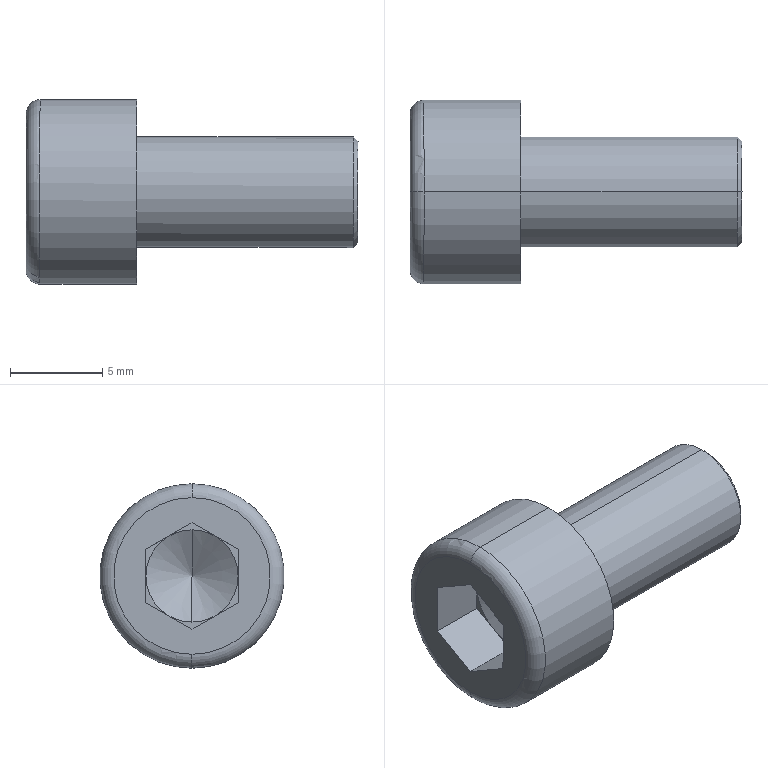Component | SolidWorks | hexagon socket head cap screws gb-88 | 1 solid | 25 faces | box 18.01 x 10 x 10.01 mm | volume 732 mm3 | plane 15 | cone 4 | cylinder 4 | torus 2 | commonest cylinder face diameters 6 x2 10 x2
STEP:
#1=COLOUR_RGB('',0.7922,0.8196,0.9333);
#2=FILL_AREA_STYLE_COLOUR('',#1);
#3=FILL_AREA_STYLE('',(#2));
#4=SURFACE_STYLE_FILL_AREA(#3);
#5=SURFACE_SIDE_STYLE('',(#4));
#6=SURFACE_STYLE_USAGE(.BOTH.,#5);
#7=PRESENTATION_STYLE_ASSIGNMENT((#6));
#8=CARTESIAN_POINT('',(-2.934,36.006,44.762));
#9=VERTEX_POINT('',#8);
#10=CARTESIAN_POINT('',(-2.933,36.006,44.978));
#11=VERTEX_POINT('',#10);
#12=CARTESIAN_POINT('',(-2.933,36.006,44.87));
#13=DIRECTION('',(1.,0.,-0.00108));
#14=DIRECTION('',(-0.00108,0.,-1.));
#15=AXIS2_PLACEMENT_3D('',#12,#13,#14);
#16=CIRCLE('',#15,0.1083);
#17=EDGE_CURVE('',#9,#11,#16,.T.);
#18=ORIENTED_EDGE('',*,*,#17,.F.);
#19=CARTESIAN_POINT('',(-2.943,36.006,44.752));
#20=VERTEX_POINT('',#19);
#21=CARTESIAN_POINT('',(-2.934,36.006,44.762));
#22=DIRECTION('',(-0.7079,0.,-0.7063));
#23=VECTOR('',#22,39.37);
#24=LINE('',#21,#23);
#25=EDGE_CURVE('',#9,#20,#24,.T.);
#26=ORIENTED_EDGE('',*,*,#25,.T.);
#27=CARTESIAN_POINT('',(-2.943,36.006,44.988));
#28=VERTEX_POINT('',#27);
#29=CARTESIAN_POINT('',(-2.943,36.006,44.87));
#30=DIRECTION('',(-1.,-0.,0.00108));
#31=DIRECTION('',(-0.00108,0.,-1.));
#32=AXIS2_PLACEMENT_3D('',#29,#30,#31);
#33=CIRCLE('',#32,0.1181);
#34=EDGE_CURVE('',#28,#20,#33,.T.);
#35=ORIENTED_EDGE('',*,*,#34,.F.);
#36=CARTESIAN_POINT('',(-2.933,36.006,44.978));
#37=DIRECTION('',(-0.7063,-0.,0.7079));
#38=VECTOR('',#37,39.37);
#39=LINE('',#36,#38);
#40=EDGE_CURVE('',#11,#28,#39,.T.);
#41=ORIENTED_EDGE('',*,*,#40,.F.);
#42=EDGE_LOOP('',(#18,#26,#35,#41));
#43=FACE_OUTER_BOUND('',#42,.T.);
#44=CARTESIAN_POINT('',(-2.933,36.006,44.87));
#45=DIRECTION('',(-1.,-0.,0.00108));
#46=DIRECTION('',(0.00108,-0.,1.));
#47=AXIS2_PLACEMENT_3D('',#44,#45,#46);
#48=CONICAL_SURFACE('',#47,0.1083,0.7854);
#49=ADVANCED_FACE('',(#43),#48,.T.);
#50=CARTESIAN_POINT('',(-3.642,36.006,45.038));
#51=VERTEX_POINT('',#50);
#52=CARTESIAN_POINT('',(-3.642,36.006,44.703));
#53=VERTEX_POINT('',#52);
#54=CARTESIAN_POINT('',(-3.642,36.006,44.871));
#55=DIRECTION('',(-1.,-0.,0.00108));
#56=DIRECTION('',(-0.00108,0.,-1.));
#57=AXIS2_PLACEMENT_3D('',#54,#55,#56);
#58=CIRCLE('',#57,0.1673);
#59=EDGE_CURVE('',#51,#53,#58,.T.);
#60=ORIENTED_EDGE('',*,*,#59,.F.);
#61=CARTESIAN_POINT('',(-3.612,36.006,45.068));
#62=VERTEX_POINT('',#61);
#63=CARTESIAN_POINT('',(-3.612,36.006,45.038));
#64=DIRECTION('',(0.,1.,0.));
#65=DIRECTION('',(0.,-0.,1.));
#66=AXIS2_PLACEMENT_3D('',#63,#64,#65);
#67=CIRCLE('',#66,0.02953);
#68=EDGE_CURVE('',#51,#62,#67,.T.);
#69=ORIENTED_EDGE('',*,*,#68,.T.);
#70=CARTESIAN_POINT('',(-3.613,36.006,44.674));
#71=VERTEX_POINT('',#70);
#72=CARTESIAN_POINT('',(-3.613,36.006,44.871));
#73=DIRECTION('',(1.,0.,-0.00108));
#74=DIRECTION('',(-0.00108,0.,-1.));
#75=AXIS2_PLACEMENT_3D('',#72,#73,#74);
#76=CIRCLE('',#75,0.1969);
#77=EDGE_CURVE('',#71,#62,#76,.T.);
#78=ORIENTED_EDGE('',*,*,#77,.F.);
#79=CARTESIAN_POINT('',(-3.613,36.006,44.703));
#80=DIRECTION('',(-0.,-1.,-0.));
#81=DIRECTION('',(0.,0.,-1.));
#82=AXIS2_PLACEMENT_3D('',#79,#80,#81);
#83=CIRCLE('',#82,0.02953);
#84=EDGE_CURVE('',#53,#71,#83,.T.);
#85=ORIENTED_EDGE('',*,*,#84,.F.);
#86=EDGE_LOOP('',(#60,#69,#78,#85));
#87=FACE_OUTER_BOUND('',#86,.T.);
#88=CARTESIAN_POINT('',(-3.613,36.006,44.871));
#89=DIRECTION('',(1.,0.,-0.00108));
#90=DIRECTION('',(-0.00108,0.,-1.));
#91=AXIS2_PLACEMENT_3D('',#88,#89,#90);
#92=TOROIDAL_SURFACE('',#91,0.1673,0.02953);
#93=ADVANCED_FACE('',(#87),#92,.T.);
#94=CARTESIAN_POINT('',(-3.467,36.006,44.871));
#95=VERTEX_POINT('',#94);
#96=CARTESIAN_POINT('',(-3.524,36.006,44.969));
#97=VERTEX_POINT('',#96);
#98=CARTESIAN_POINT('',(-3.524,36.006,44.969));
#99=DIRECTION('',(-0.4991,-0.,0.8666));
#100=VECTOR('',#99,39.37);
#101=LINE('',#98,#100);
#102=EDGE_CURVE('',#95,#97,#101,.T.);
#103=ORIENTED_EDGE('',*,*,#102,.F.);
#104=CARTESIAN_POINT('',(-3.524,36.006,44.772));
#105=VERTEX_POINT('',#104);
#106=CARTESIAN_POINT('',(-3.524,36.006,44.772));
#107=DIRECTION('',(-0.5009,0.,-0.8655));
#108=VECTOR('',#107,39.37);
#109=LINE('',#106,#108);
#110=EDGE_CURVE('',#95,#105,#109,.T.);
#111=ORIENTED_EDGE('',*,*,#110,.T.);
#112=CARTESIAN_POINT('',(-3.524,35.956,44.785));
#113=VERTEX_POINT('',#112);
#114=CARTESIAN_POINT('',(-3.524,36.006,44.871));
#115=DIRECTION('',(-1.,-0.,0.00108));
#116=DIRECTION('',(-0.00108,0.,-1.));
#117=AXIS2_PLACEMENT_3D('',#114,#115,#116);
#118=CIRCLE('',#117,0.09843);
#119=EDGE_CURVE('',#105,#113,#118,.T.);
#120=ORIENTED_EDGE('',*,*,#119,.T.);
#121=CARTESIAN_POINT('',(-3.524,35.907,44.871));
#122=VERTEX_POINT('',#121);
#123=CARTESIAN_POINT('',(-3.524,36.006,44.871));
#124=DIRECTION('',(-1.,-0.,0.00108));
#125=DIRECTION('',(-0.00108,0.,-1.));
#126=AXIS2_PLACEMENT_3D('',#123,#124,#125);
#127=CIRCLE('',#126,0.09843);
#128=EDGE_CURVE('',#113,#122,#127,.T.);
#129=ORIENTED_EDGE('',*,*,#128,.T.);
#130=CARTESIAN_POINT('',(-3.524,35.956,44.956));
#131=VERTEX_POINT('',#130);
#132=CARTESIAN_POINT('',(-3.524,36.006,44.871));
#133=DIRECTION('',(-1.,-0.,0.00108));
#134=DIRECTION('',(-0.00108,0.,-1.));
#135=AXIS2_PLACEMENT_3D('',#132,#133,#134);
#136=CIRCLE('',#135,0.09843);
#137=EDGE_CURVE('',#122,#131,#136,.T.);
#138=ORIENTED_EDGE('',*,*,#137,.T.);
#139=CARTESIAN_POINT('',(-3.524,36.006,44.871));
#140=DIRECTION('',(-1.,-0.,0.00108));
#141=DIRECTION('',(-0.00108,0.,-1.));
#142=AXIS2_PLACEMENT_3D('',#139,#140,#141);
#143=CIRCLE('',#142,0.09843);
#144=EDGE_CURVE('',#131,#97,#143,.T.);
#145=ORIENTED_EDGE('',*,*,#144,.T.);
#146=EDGE_LOOP('',(#103,#111,#120,#129,#138,#145));
#147=FACE_OUTER_BOUND('',#146,.T.);
#148=CARTESIAN_POINT('',(-3.524,36.006,44.871));
#149=DIRECTION('',(-1.,-0.,0.00108));
#150=DIRECTION('',(0.00108,-0.,1.));
#151=AXIS2_PLACEMENT_3D('',#148,#149,#150);
#152=CONICAL_SURFACE('',#151,0.09843,1.047);
#153=ADVANCED_FACE('',(#147),#152,.F.);
#154=ORIENTED_EDGE('',*,*,#34,.T.);
#155=CARTESIAN_POINT('',(-3.406,36.006,44.752));
#156=VERTEX_POINT('',#155);
#157=CARTESIAN_POINT('',(-2.934,36.006,44.752));
#158=DIRECTION('',(-1.,-0.,0.00108));
#159=VECTOR('',#158,39.37);
#160=LINE('',#157,#159);
#161=EDGE_CURVE('',#20,#156,#160,.T.);
#162=ORIENTED_EDGE('',*,*,#161,.T.);
#163=CARTESIAN_POINT('',(-3.406,36.006,44.989));
#164=VERTEX_POINT('',#163);
#165=CARTESIAN_POINT('',(-3.406,36.006,44.871));
#166=DIRECTION('',(1.,0.,-0.00108));
#167=DIRECTION('',(-0.00108,0.,-1.));
#168=AXIS2_PLACEMENT_3D('',#165,#166,#167);
#169=CIRCLE('',#168,0.1181);
#170=EDGE_CURVE('',#156,#164,#169,.T.);
#171=ORIENTED_EDGE('',*,*,#170,.T.);
#172=CARTESIAN_POINT('',(-2.933,36.006,44.988));
#173=DIRECTION('',(-1.,-0.,0.00108));
#174=VECTOR('',#173,39.37);
#175=LINE('',#172,#174);
#176=EDGE_CURVE('',#28,#164,#175,.T.);
#177=ORIENTED_EDGE('',*,*,#176,.F.);
#178=EDGE_LOOP('',(#154,#162,#171,#177));
#179=FACE_OUTER_BOUND('',#178,.T.);
#180=CARTESIAN_POINT('',(-2.933,36.006,44.87));
#181=DIRECTION('',(-1.,-0.,0.00108));
#182=DIRECTION('',(0.00108,-0.,1.));
#183=AXIS2_PLACEMENT_3D('',#180,#181,#182);
#184=CYLINDRICAL_SURFACE('',#183,0.1181);
#185=ADVANCED_FACE('',(#179),#184,.T.);
#186=CARTESIAN_POINT('',(-3.406,36.006,44.674));
#187=VERTEX_POINT('',#186);
#188=CARTESIAN_POINT('',(-3.406,36.006,45.067));
#189=VERTEX_POINT('',#188);
#190=CARTESIAN_POINT('',(-3.406,36.006,44.871));
#191=DIRECTION('',(1.,0.,-0.00108));
#192=DIRECTION('',(-0.00108,0.,-1.));
#193=AXIS2_PLACEMENT_3D('',#190,#191,#192);
#194=CIRCLE('',#193,0.1969);
#195=EDGE_CURVE('',#187,#189,#194,.T.);
#196=ORIENTED_EDGE('',*,*,#195,.F.);
#197=CARTESIAN_POINT('',(-3.406,36.006,44.674));
#198=DIRECTION('',(-1.,-0.,0.00108));
#199=VECTOR('',#198,39.37);
#200=LINE('',#197,#199);
#201=EDGE_CURVE('',#187,#71,#200,.T.);
#202=ORIENTED_EDGE('',*,*,#201,.T.);
#203=ORIENTED_EDGE('',*,*,#77,.T.);
#204=CARTESIAN_POINT('',(-3.406,36.006,45.067));
#205=DIRECTION('',(-1.,-0.,0.00108));
#206=VECTOR('',#205,39.37);
#207=LINE('',#204,#206);
#208=EDGE_CURVE('',#189,#62,#207,.T.);
#209=ORIENTED_EDGE('',*,*,#208,.F.);
#210=EDGE_LOOP('',(#196,#202,#203,#209));
#211=FACE_OUTER_BOUND('',#210,.T.);
#212=CARTESIAN_POINT('',(-3.406,36.006,44.871));
#213=DIRECTION('',(-1.,-0.,0.00108));
#214=DIRECTION('',(0.00108,-0.,1.));
#215=AXIS2_PLACEMENT_3D('',#212,#213,#214);
#216=CYLINDRICAL_SURFACE('',#215,0.1969);
#217=ADVANCED_FACE('',(#211),#216,.T.);
#218=ORIENTED_EDGE('',*,*,#128,.F.);
#219=CARTESIAN_POINT('',(-3.524,35.907,44.814));
#220=VERTEX_POINT('',#219);
#221=CARTESIAN_POINT('',(-3.524,35.907,44.814));
#222=DIRECTION('',(-0.0005402,0.866,-0.5));
#223=VECTOR('',#222,39.37);
#224=LINE('',#221,#223);
#225=EDGE_CURVE('',#220,#113,#224,.T.);
#226=ORIENTED_EDGE('',*,*,#225,.F.);
#227=CARTESIAN_POINT('',(-3.524,35.907,44.927));
#228=DIRECTION('',(-0.00108,0.,-1.));
#229=VECTOR('',#228,39.37);
#230=LINE('',#227,#229);
#231=EDGE_CURVE('',#122,#220,#230,.T.);
#232=ORIENTED_EDGE('',*,*,#231,.F.);
#233=EDGE_LOOP('',(#218,#226,#232));
#234=FACE_OUTER_BOUND('',#233,.T.);
#235=CARTESIAN_POINT('',(-3.524,36.006,44.757));
#236=DIRECTION('',(1.,0.,-0.00108));
#237=DIRECTION('',(-0.00108,0.,-1.));
#238=AXIS2_PLACEMENT_3D('',#235,#236,#237);
#239=PLANE('',#238);
#240=ADVANCED_FACE('',(#234),#239,.F.);
#241=ORIENTED_EDGE('',*,*,#137,.F.);
#242=CARTESIAN_POINT('',(-3.524,35.907,44.927));
#243=VERTEX_POINT('',#242);
#244=CARTESIAN_POINT('',(-3.524,35.907,44.927));
#245=DIRECTION('',(-0.00108,0.,-1.));
#246=VECTOR('',#245,39.37);
#247=LINE('',#244,#246);
#248=EDGE_CURVE('',#243,#122,#247,.T.);
#249=ORIENTED_EDGE('',*,*,#248,.F.);
#250=CARTESIAN_POINT('',(-3.524,36.006,44.984));
#251=DIRECTION('',(-0.0005402,-0.866,-0.5));
#252=VECTOR('',#251,39.37);
#253=LINE('',#250,#252);
#254=EDGE_CURVE('',#131,#243,#253,.T.);
#255=ORIENTED_EDGE('',*,*,#254,.F.);
#256=EDGE_LOOP('',(#241,#249,#255));
#257=FACE_OUTER_BOUND('',#256,.T.);
#258=CARTESIAN_POINT('',(-3.524,36.006,44.757));
#259=DIRECTION('',(1.,0.,-0.00108));
#260=DIRECTION('',(-0.00108,0.,-1.));
#261=AXIS2_PLACEMENT_3D('',#258,#259,#260);
#262=PLANE('',#261);
#263=ADVANCED_FACE('',(#257),#262,.F.);
#264=ORIENTED_EDGE('',*,*,#144,.F.);
#265=CARTESIAN_POINT('',(-3.524,36.006,44.984));
#266=VERTEX_POINT('',#265);
#267=CARTESIAN_POINT('',(-3.524,36.006,44.984));
#268=DIRECTION('',(-0.0005402,-0.866,-0.5));
#269=VECTOR('',#268,39.37);
#270=LINE('',#267,#269);
#271=EDGE_CURVE('',#266,#131,#270,.T.);
#272=ORIENTED_EDGE('',*,*,#271,.F.);
#273=CARTESIAN_POINT('',(-3.524,36.055,44.956));
#274=VERTEX_POINT('',#273);
#275=CARTESIAN_POINT('',(-3.524,36.104,44.927));
#276=DIRECTION('',(0.0005402,-0.866,0.5));
#277=VECTOR('',#276,39.37);
#278=LINE('',#275,#277);
#279=EDGE_CURVE('',#274,#266,#278,.T.);
#280=ORIENTED_EDGE('',*,*,#279,.F.);
#281=CARTESIAN_POINT('',(-3.524,36.006,44.871));
#282=DIRECTION('',(-1.,-0.,0.00108));
#283=DIRECTION('',(-0.00108,0.,-1.));
#284=AXIS2_PLACEMENT_3D('',#281,#282,#283);
#285=CIRCLE('',#284,0.09843);
#286=EDGE_CURVE('',#97,#274,#285,.T.);
#287=ORIENTED_EDGE('',*,*,#286,.F.);
#288=EDGE_LOOP('',(#264,#272,#280,#287));
#289=FACE_OUTER_BOUND('',#288,.T.);
#290=CARTESIAN_POINT('',(-3.524,36.006,44.757));
#291=DIRECTION('',(1.,0.,-0.00108));
#292=DIRECTION('',(-0.00108,0.,-1.));
#293=AXIS2_PLACEMENT_3D('',#290,#291,#292);
#294=PLANE('',#293);
#295=ADVANCED_FACE('',(#289),#294,.F.);
#296=CARTESIAN_POINT('',(-3.524,36.104,44.871));
#297=VERTEX_POINT('',#296);
#298=CARTESIAN_POINT('',(-3.524,36.006,44.871));
#299=DIRECTION('',(-1.,-0.,0.00108));
#300=DIRECTION('',(-0.00108,0.,-1.));
#301=AXIS2_PLACEMENT_3D('',#298,#299,#300);
#302=CIRCLE('',#301,0.09843);
#303=EDGE_CURVE('',#274,#297,#302,.T.);
#304=ORIENTED_EDGE('',*,*,#303,.F.);
#305=CARTESIAN_POINT('',(-3.524,36.104,44.927));
#306=VERTEX_POINT('',#305);
#307=CARTESIAN_POINT('',(-3.524,36.104,44.927));
#308=DIRECTION('',(0.0005402,-0.866,0.5));
#309=VECTOR('',#308,39.37);
#310=LINE('',#307,#309);
#311=EDGE_CURVE('',#306,#274,#310,.T.);
#312=ORIENTED_EDGE('',*,*,#311,.F.);
#313=CARTESIAN_POINT('',(-3.524,36.104,44.814));
#314=DIRECTION('',(0.00108,-0.,1.));
#315=VECTOR('',#314,39.37);
#316=LINE('',#313,#315);
#317=EDGE_CURVE('',#297,#306,#316,.T.);
#318=ORIENTED_EDGE('',*,*,#317,.F.);
#319=EDGE_LOOP('',(#304,#312,#318));
#320=FACE_OUTER_BOUND('',#319,.T.);
#321=CARTESIAN_POINT('',(-3.524,36.006,44.757));
#322=DIRECTION('',(1.,0.,-0.00108));
#323=DIRECTION('',(-0.00108,0.,-1.));
#324=AXIS2_PLACEMENT_3D('',#321,#322,#323);
#325=PLANE('',#324);
#326=ADVANCED_FACE('',(#320),#325,.F.);
#327=CARTESIAN_POINT('',(-3.524,36.055,44.785));
#328=VERTEX_POINT('',#327);
#329=CARTESIAN_POINT('',(-3.524,36.006,44.871));
#330=DIRECTION('',(1.,0.,-0.00108));
#331=DIRECTION('',(-0.00108,0.,-1.));
#332=AXIS2_PLACEMENT_3D('',#329,#330,#331);
#333=CIRCLE('',#332,0.09843);
#334=EDGE_CURVE('',#328,#297,#333,.T.);
#335=ORIENTED_EDGE('',*,*,#334,.T.);
#336=CARTESIAN_POINT('',(-3.524,36.104,44.814));
#337=VERTEX_POINT('',#336);
#338=CARTESIAN_POINT('',(-3.524,36.104,44.814));
#339=DIRECTION('',(0.00108,-0.,1.));
#340=VECTOR('',#339,39.37);
#341=LINE('',#338,#340);
#342=EDGE_CURVE('',#337,#297,#341,.T.);
#343=ORIENTED_EDGE('',*,*,#342,.F.);
#344=CARTESIAN_POINT('',(-3.524,36.006,44.757));
#345=DIRECTION('',(0.0005402,0.866,0.5));
#346=VECTOR('',#345,39.37);
#347=LINE('',#344,#346);
#348=EDGE_CURVE('',#328,#337,#347,.T.);
#349=ORIENTED_EDGE('',*,*,#348,.F.);
#350=EDGE_LOOP('',(#335,#343,#349));
#351=FACE_OUTER_BOUND('',#350,.T.);
#352=CARTESIAN_POINT('',(-3.524,36.006,44.757));
#353=DIRECTION('',(1.,0.,-0.00108));
#354=DIRECTION('',(-0.00108,0.,-1.));
#355=AXIS2_PLACEMENT_3D('',#352,#353,#354);
#356=PLANE('',#355);
#357=ADVANCED_FACE('',(#351),#356,.F.);
#358=CARTESIAN_POINT('',(-3.524,36.006,44.871));
#359=DIRECTION('',(-1.,-0.,0.00108));
#360=DIRECTION('',(-0.00108,0.,-1.));
#361=AXIS2_PLACEMENT_3D('',#358,#359,#360);
#362=CIRCLE('',#361,0.09843);
#363=EDGE_CURVE('',#328,#105,#362,.T.);
#364=ORIENTED_EDGE('',*,*,#363,.F.);
#365=CARTESIAN_POINT('',(-3.524,36.006,44.757));
#366=VERTEX_POINT('',#365);
#367=CARTESIAN_POINT('',(-3.524,36.006,44.757));
#368=DIRECTION('',(0.0005402,0.866,0.5));
#369=VECTOR('',#368,39.37);
#370=LINE('',#367,#369);
#371=EDGE_CURVE('',#366,#328,#370,.T.);
#372=ORIENTED_EDGE('',*,*,#371,.F.);
#373=CARTESIAN_POINT('',(-3.524,35.907,44.814));
#374=DIRECTION('',(-0.0005402,0.866,-0.5));
#375=VECTOR('',#374,39.37);
#376=LINE('',#373,#375);
#377=EDGE_CURVE('',#113,#366,#376,.T.);
#378=ORIENTED_EDGE('',*,*,#377,.F.);
#379=ORIENTED_EDGE('',*,*,#119,.F.);
#380=EDGE_LOOP('',(#364,#372,#378,#379));
#381=FACE_OUTER_BOUND('',#380,.T.);
#382=CARTESIAN_POINT('',(-3.524,36.006,44.757));
#383=DIRECTION('',(1.,0.,-0.00108));
#384=DIRECTION('',(-0.00108,0.,-1.));
#385=AXIS2_PLACEMENT_3D('',#382,#383,#384);
#386=PLANE('',#385);
#387=ADVANCED_FACE('',(#381),#386,.F.);
#388=CARTESIAN_POINT('',(-3.642,36.006,44.871));
#389=DIRECTION('',(-1.,-0.,0.00108));
#390=DIRECTION('',(-0.00108,0.,-1.));
#391=AXIS2_PLACEMENT_3D('',#388,#389,#390);
#392=CIRCLE('',#391,0.1673);
#393=EDGE_CURVE('',#53,#51,#392,.T.);
#394=ORIENTED_EDGE('',*,*,#393,.T.);
#395=ORIENTED_EDGE('',*,*,#59,.T.);
#396=EDGE_LOOP('',(#394,#395));
#397=FACE_OUTER_BOUND('',#396,.T.);
#398=CARTESIAN_POINT('',(-3.642,35.907,44.814));
#399=VERTEX_POINT('',#398);
#400=CARTESIAN_POINT('',(-3.642,36.006,44.757));
#401=VERTEX_POINT('',#400);
#402=CARTESIAN_POINT('',(-3.642,35.907,44.814));
#403=DIRECTION('',(-0.0005402,0.866,-0.5));
#404=VECTOR('',#403,39.37);
#405=LINE('',#402,#404);
#406=EDGE_CURVE('',#399,#401,#405,.T.);
#407=ORIENTED_EDGE('',*,*,#406,.T.);
#408=CARTESIAN_POINT('',(-3.642,36.104,44.814));
#409=VERTEX_POINT('',#408);
#410=CARTESIAN_POINT('',(-3.642,36.006,44.757));
#411=DIRECTION('',(0.0005402,0.866,0.5));
#412=VECTOR('',#411,39.37);
#413=LINE('',#410,#412);
#414=EDGE_CURVE('',#401,#409,#413,.T.);
#415=ORIENTED_EDGE('',*,*,#414,.T.);
#416=CARTESIAN_POINT('',(-3.642,36.104,44.928));
#417=VERTEX_POINT('',#416);
#418=CARTESIAN_POINT('',(-3.642,36.104,44.814));
#419=DIRECTION('',(0.00108,-0.,1.));
#420=VECTOR('',#419,39.37);
#421=LINE('',#418,#420);
#422=EDGE_CURVE('',#409,#417,#421,.T.);
#423=ORIENTED_EDGE('',*,*,#422,.T.);
#424=CARTESIAN_POINT('',(-3.642,36.006,44.984));
#425=VERTEX_POINT('',#424);
#426=CARTESIAN_POINT('',(-3.642,36.104,44.928));
#427=DIRECTION('',(0.0005402,-0.866,0.5));
#428=VECTOR('',#427,39.37);
#429=LINE('',#426,#428);
#430=EDGE_CURVE('',#417,#425,#429,.T.);
#431=ORIENTED_EDGE('',*,*,#430,.T.);
#432=CARTESIAN_POINT('',(-3.642,35.907,44.928));
#433=VERTEX_POINT('',#432);
#434=CARTESIAN_POINT('',(-3.642,36.006,44.984));
#435=DIRECTION('',(-0.0005402,-0.866,-0.5));
#436=VECTOR('',#435,39.37);
#437=LINE('',#434,#436);
#438=EDGE_CURVE('',#425,#433,#437,.T.);
#439=ORIENTED_EDGE('',*,*,#438,.T.);
#440=CARTESIAN_POINT('',(-3.642,35.907,44.928));
#441=DIRECTION('',(-0.00108,0.,-1.));
#442=VECTOR('',#441,39.37);
#443=LINE('',#440,#442);
#444=EDGE_CURVE('',#433,#399,#443,.T.);
#445=ORIENTED_EDGE('',*,*,#444,.T.);
#446=EDGE_LOOP('',(#407,#415,#423,#431,#439,#445));
#447=FACE_BOUND('',#446,.T.);
#448=CARTESIAN_POINT('',(-3.642,36.006,44.871));
#449=DIRECTION('',(1.,0.,-0.00108));
#450=DIRECTION('',(-0.00108,0.,-1.));
#451=AXIS2_PLACEMENT_3D('',#448,#449,#450);
#452=PLANE('',#451);
#453=ADVANCED_FACE('',(#397,#447),#452,.F.);
#454=CARTESIAN_POINT('',(-3.406,36.006,44.871));
#455=DIRECTION('',(1.,0.,-0.00108));
#456=DIRECTION('',(-0.00108,0.,-1.));
#457=AXIS2_PLACEMENT_3D('',#454,#455,#456);
#458=CIRCLE('',#457,0.1969);
#459=EDGE_CURVE('',#189,#187,#458,.T.);
#460=ORIENTED_EDGE('',*,*,#459,.T.);
#461=ORIENTED_EDGE('',*,*,#195,.T.);
#462=EDGE_LOOP('',(#460,#461));
#463=FACE_OUTER_BOUND('',#462,.T.);
#464=CARTESIAN_POINT('',(-3.406,36.006,44.871));
#465=DIRECTION('',(1.,0.,-0.00108));
#466=DIRECTION('',(-0.00108,0.,-1.));
#467=AXIS2_PLACEMENT_3D('',#464,#465,#466);
#468=CIRCLE('',#467,0.1181);
#469=EDGE_CURVE('',#164,#156,#468,.T.);
#470=ORIENTED_EDGE('',*,*,#469,.F.);
#471=ORIENTED_EDGE('',*,*,#170,.F.);
#472=EDGE_LOOP('',(#470,#471));
#473=FACE_BOUND('',#472,.T.);
#474=CARTESIAN_POINT('',(-3.406,36.006,44.871));
#475=DIRECTION('',(1.,0.,-0.00108));
#476=DIRECTION('',(-0.00108,0.,-1.));
#477=AXIS2_PLACEMENT_3D('',#474,#475,#476);
#478=PLANE('',#477);
#479=ADVANCED_FACE('',(#463,#473),#478,.T.);
#480=ORIENTED_EDGE('',*,*,#201,.F.);
#481=ORIENTED_EDGE('',*,*,#459,.F.);
#482=ORIENTED_EDGE('',*,*,#208,.T.);
#483=CARTESIAN_POINT('',(-3.613,36.006,44.871));
#484=DIRECTION('',(1.,0.,-0.00108));
#485=DIRECTION('',(-0.00108,0.,-1.));
#486=AXIS2_PLACEMENT_3D('',#483,#484,#485);
#487=CIRCLE('',#486,0.1969);
#488=EDGE_CURVE('',#62,#71,#487,.T.);
#489=ORIENTED_EDGE('',*,*,#488,.T.);
#490=EDGE_LOOP('',(#480,#481,#482,#489));
#491=FACE_OUTER_BOUND('',#490,.T.);
#492=CARTESIAN_POINT('',(-3.406,36.006,44.871));
#493=DIRECTION('',(-1.,-0.,0.00108));
#494=DIRECTION('',(0.00108,-0.,1.));
#495=AXIS2_PLACEMENT_3D('',#492,#493,#494);
#496=CYLINDRICAL_SURFACE('',#495,0.1969);
#497=ADVANCED_FACE('',(#491),#496,.T.);
#498=ORIENTED_EDGE('',*,*,#161,.F.);
#499=CARTESIAN_POINT('',(-2.943,36.006,44.87));
#500=DIRECTION('',(-1.,-0.,0.00108));
#501=DIRECTION('',(-0.00108,0.,-1.));
#502=AXIS2_PLACEMENT_3D('',#499,#500,#501);
#503=CIRCLE('',#502,0.1181);
#504=EDGE_CURVE('',#20,#28,#503,.T.);
#505=ORIENTED_EDGE('',*,*,#504,.T.);
#506=ORIENTED_EDGE('',*,*,#176,.T.);
#507=ORIENTED_EDGE('',*,*,#469,.T.);
#508=EDGE_LOOP('',(#498,#505,#506,#507));
#509=FACE_OUTER_BOUND('',#508,.T.);
#510=CARTESIAN_POINT('',(-2.933,36.006,44.87));
#511=DIRECTION('',(-1.,-0.,0.00108));
#512=DIRECTION('',(0.00108,-0.,1.));
#513=AXIS2_PLACEMENT_3D('',#510,#511,#512);
#514=CYLINDRICAL_SURFACE('',#513,0.1181);
#515=ADVANCED_FACE('',(#509),#514,.T.);
#516=CARTESIAN_POINT('',(-2.933,36.006,44.87));
#517=DIRECTION('',(1.,0.,-0.00108));
#518=DIRECTION('',(-0.00108,0.,-1.));
#519=AXIS2_PLACEMENT_3D('',#516,#517,#518);
#520=CIRCLE('',#519,0.1083);
#521=EDGE_CURVE('',#11,#9,#520,.T.);
#522=ORIENTED_EDGE('',*,*,#521,.T.);
#523=ORIENTED_EDGE('',*,*,#17,.T.);
#524=EDGE_LOOP('',(#522,#523));
#525=FACE_OUTER_BOUND('',#524,.T.);
#526=CARTESIAN_POINT('',(-2.933,36.006,44.87));
#527=DIRECTION('',(1.,0.,-0.00108));
#528=DIRECTION('',(-0.00108,0.,-1.));
#529=AXIS2_PLACEMENT_3D('',#526,#527,#528);
#530=PLANE('',#529);
#531=ADVANCED_FACE('',(#525),#530,.T.);
#532=ORIENTED_EDGE('',*,*,#406,.F.);
#533=CARTESIAN_POINT('',(-3.524,35.907,44.814));
#534=DIRECTION('',(-1.,-0.,0.00108));
#535=VECTOR('',#534,39.37);
#536=LINE('',#533,#535);
#537=EDGE_CURVE('',#220,#399,#536,.T.);
#538=ORIENTED_EDGE('',*,*,#537,.F.);
#539=ORIENTED_EDGE('',*,*,#225,.T.);
#540=ORIENTED_EDGE('',*,*,#377,.T.);
#541=CARTESIAN_POINT('',(-3.524,36.006,44.757));
#542=DIRECTION('',(-1.,-0.,0.00108));
#543=VECTOR('',#542,39.37);
#544=LINE('',#541,#543);
#545=EDGE_CURVE('',#366,#401,#544,.T.);
#546=ORIENTED_EDGE('',*,*,#545,.T.);
#547=EDGE_LOOP('',(#532,#538,#539,#540,#546));
#548=FACE_OUTER_BOUND('',#547,.T.);
#549=CARTESIAN_POINT('',(-3.524,35.907,44.814));
#550=DIRECTION('',(0.0009357,0.5,0.866));
#551=DIRECTION('',(0.0005402,-0.866,0.5));
#552=AXIS2_PLACEMENT_3D('',#549,#550,#551);
#553=PLANE('',#552);
#554=ADVANCED_FACE('',(#548),#553,.T.);
#555=ORIENTED_EDGE('',*,*,#414,.F.);
#556=ORIENTED_EDGE('',*,*,#545,.F.);
#557=ORIENTED_EDGE('',*,*,#371,.T.);
#558=ORIENTED_EDGE('',*,*,#348,.T.);
#559=CARTESIAN_POINT('',(-3.524,36.104,44.814));
#560=DIRECTION('',(-1.,-0.,0.00108));
#561=VECTOR('',#560,39.37);
#562=LINE('',#559,#561);
#563=EDGE_CURVE('',#337,#409,#562,.T.);
#564=ORIENTED_EDGE('',*,*,#563,.T.);
#565=EDGE_LOOP('',(#555,#556,#557,#558,#564));
#566=FACE_OUTER_BOUND('',#565,.T.);
#567=CARTESIAN_POINT('',(-3.524,36.006,44.757));
#568=DIRECTION('',(0.0009357,-0.5,0.866));
#569=DIRECTION('',(-0.0005402,-0.866,-0.5));
#570=AXIS2_PLACEMENT_3D('',#567,#568,#569);
#571=PLANE('',#570);
#572=ADVANCED_FACE('',(#566),#571,.T.);
#573=ORIENTED_EDGE('',*,*,#422,.F.);
#574=ORIENTED_EDGE('',*,*,#563,.F.);
#575=ORIENTED_EDGE('',*,*,#342,.T.);
#576=ORIENTED_EDGE('',*,*,#317,.T.);
#577=CARTESIAN_POINT('',(-3.524,36.104,44.927));
#578=DIRECTION('',(-1.,-0.,0.00108));
#579=VECTOR('',#578,39.37);
#580=LINE('',#577,#579);
#581=EDGE_CURVE('',#306,#417,#580,.T.);
#582=ORIENTED_EDGE('',*,*,#581,.T.);
#583=EDGE_LOOP('',(#573,#574,#575,#576,#582));
#584=FACE_OUTER_BOUND('',#583,.T.);
#585=CARTESIAN_POINT('',(-3.524,36.104,44.814));
#586=DIRECTION('',(-0.,-1.,-0.));
#587=DIRECTION('',(-0.00108,0.,-1.));
#588=AXIS2_PLACEMENT_3D('',#585,#586,#587);
#589=PLANE('',#588);
#590=ADVANCED_FACE('',(#584),#589,.T.);
#591=ORIENTED_EDGE('',*,*,#430,.F.);
#592=ORIENTED_EDGE('',*,*,#581,.F.);
#593=ORIENTED_EDGE('',*,*,#311,.T.);
#594=ORIENTED_EDGE('',*,*,#279,.T.);
#595=CARTESIAN_POINT('',(-3.524,36.006,44.984));
#596=DIRECTION('',(-1.,-0.,0.00108));
#597=VECTOR('',#596,39.37);
#598=LINE('',#595,#597);
#599=EDGE_CURVE('',#266,#425,#598,.T.);
#600=ORIENTED_EDGE('',*,*,#599,.T.);
#601=EDGE_LOOP('',(#591,#592,#593,#594,#600));
#602=FACE_OUTER_BOUND('',#601,.T.);
#603=CARTESIAN_POINT('',(-3.524,36.104,44.927));
#604=DIRECTION('',(-0.0009357,-0.5,-0.866));
#605=DIRECTION('',(-0.0005402,0.866,-0.5));
#606=AXIS2_PLACEMENT_3D('',#603,#604,#605);
#607=PLANE('',#606);
#608=ADVANCED_FACE('',(#602),#607,.T.);
#609=ORIENTED_EDGE('',*,*,#438,.F.);
#610=ORIENTED_EDGE('',*,*,#599,.F.);
#611=ORIENTED_EDGE('',*,*,#271,.T.);
#612=ORIENTED_EDGE('',*,*,#254,.T.);
#613=CARTESIAN_POINT('',(-3.524,35.907,44.927));
#614=DIRECTION('',(-1.,-0.,0.00108));
#615=VECTOR('',#614,39.37);
#616=LINE('',#613,#615);
#617=EDGE_CURVE('',#243,#433,#616,.T.);
#618=ORIENTED_EDGE('',*,*,#617,.T.);
#619=EDGE_LOOP('',(#609,#610,#611,#612,#618));
#620=FACE_OUTER_BOUND('',#619,.T.);
#621=CARTESIAN_POINT('',(-3.524,36.006,44.984));
#622=DIRECTION('',(-0.0009357,0.5,-0.866));
#623=DIRECTION('',(0.0005402,0.866,0.5));
#624=AXIS2_PLACEMENT_3D('',#621,#622,#623);
#625=PLANE('',#624);
#626=ADVANCED_FACE('',(#620),#625,.T.);
#627=ORIENTED_EDGE('',*,*,#444,.F.);
#628=ORIENTED_EDGE('',*,*,#617,.F.);
#629=ORIENTED_EDGE('',*,*,#248,.T.);
#630=ORIENTED_EDGE('',*,*,#231,.T.);
#631=ORIENTED_EDGE('',*,*,#537,.T.);
#632=EDGE_LOOP('',(#627,#628,#629,#630,#631));
#633=FACE_OUTER_BOUND('',#632,.T.);
#634=CARTESIAN_POINT('',(-3.524,35.907,44.927));
#635=DIRECTION('',(0.,1.,0.));
#636=DIRECTION('',(0.00108,-0.,1.));
#637=AXIS2_PLACEMENT_3D('',#634,#635,#636);
#638=PLANE('',#637);
#639=ADVANCED_FACE('',(#633),#638,.T.);
#640=ORIENTED_EDGE('',*,*,#110,.F.);
#641=ORIENTED_EDGE('',*,*,#102,.T.);
#642=ORIENTED_EDGE('',*,*,#286,.T.);
#643=ORIENTED_EDGE('',*,*,#303,.T.);
#644=ORIENTED_EDGE('',*,*,#334,.F.);
#645=ORIENTED_EDGE('',*,*,#363,.T.);
#646=EDGE_LOOP('',(#640,#641,#642,#643,#644,#645));
#647=FACE_OUTER_BOUND('',#646,.T.);
#648=CARTESIAN_POINT('',(-3.524,36.006,44.871));
#649=DIRECTION('',(-1.,-0.,0.00108));
#650=DIRECTION('',(0.00108,-0.,1.));
#651=AXIS2_PLACEMENT_3D('',#648,#649,#650);
#652=CONICAL_SURFACE('',#651,0.09843,1.047);
#653=ADVANCED_FACE('',(#647),#652,.F.);
#654=ORIENTED_EDGE('',*,*,#68,.F.);
#655=ORIENTED_EDGE('',*,*,#393,.F.);
#656=ORIENTED_EDGE('',*,*,#84,.T.);
#657=ORIENTED_EDGE('',*,*,#488,.F.);
#658=EDGE_LOOP('',(#654,#655,#656,#657));
#659=FACE_OUTER_BOUND('',#658,.T.);
#660=CARTESIAN_POINT('',(-3.613,36.006,44.871));
#661=DIRECTION('',(1.,0.,-0.00108));
#662=DIRECTION('',(-0.00108,0.,-1.));
#663=AXIS2_PLACEMENT_3D('',#660,#661,#662);
#664=TOROIDAL_SURFACE('',#663,0.1673,0.02953);
#665=ADVANCED_FACE('',(#659),#664,.T.);
#666=ORIENTED_EDGE('',*,*,#25,.F.);
#667=ORIENTED_EDGE('',*,*,#521,.F.);
#668=ORIENTED_EDGE('',*,*,#40,.T.);
#669=ORIENTED_EDGE('',*,*,#504,.F.);
#670=EDGE_LOOP('',(#666,#667,#668,#669));
#671=FACE_OUTER_BOUND('',#670,.T.);
#672=CARTESIAN_POINT('',(-2.933,36.006,44.87));
#673=DIRECTION('',(-1.,-0.,0.00108));
#674=DIRECTION('',(0.00108,-0.,1.));
#675=AXIS2_PLACEMENT_3D('',#672,#673,#674);
#676=CONICAL_SURFACE('',#675,0.1083,0.7854);
#677=ADVANCED_FACE('',(#671),#676,.T.);
#678=CLOSED_SHELL('',(#49,#93,#153,#185,#217,#240,#263,#295,#326,#357,#387,#453,#479,#497,#515,#531,#554,#572,#590,#608,#626,#639,#653,#665,#677));
#679=MANIFOLD_SOLID_BREP('',#678);
#680=STYLED_ITEM('',(#7),#679);
#681=(LENGTH_UNIT()NAMED_UNIT(*)SI_UNIT($,.METRE.));
#682=LENGTH_MEASURE_WITH_UNIT(LENGTH_MEASURE(0.0254),#681);
#683=DIMENSIONAL_EXPONENTS(1.,0.,0.,0.,0.,0.,0.);
#684=(CONVERSION_BASED_UNIT('',#682)LENGTH_UNIT()NAMED_UNIT(#683));
#685=UNCERTAINTY_MEASURE_WITH_UNIT(LENGTH_MEASURE(0.00001),#684,'','');
#686=(NAMED_UNIT(*)PLANE_ANGLE_UNIT()SI_UNIT($,.RADIAN.));
#687=(NAMED_UNIT(*)SI_UNIT($,.STERADIAN.)SOLID_ANGLE_UNIT());
#688=(GEOMETRIC_REPRESENTATION_CONTEXT(3)GLOBAL_UNCERTAINTY_ASSIGNED_CONTEXT((#685))GLOBAL_UNIT_ASSIGNED_CONTEXT((#684,#686,#687))REPRESENTATION_CONTEXT('',''));
#689=MECHANICAL_DESIGN_GEOMETRIC_PRESENTATION_REPRESENTATION('',(#680),#688);
#690=PRESENTATION_LAYER_ASSIGNMENT('','',(#680));
#691=CARTESIAN_POINT('',(0.,0.,0.));
#692=DIRECTION('',(0.,0.,1.));
#693=DIRECTION('',(1.,0.,0.));
#694=AXIS2_PLACEMENT_3D('',#691,#692,#693);
#695=(LENGTH_UNIT()NAMED_UNIT(*)SI_UNIT($,.METRE.));
#696=LENGTH_MEASURE_WITH_UNIT(LENGTH_MEASURE(0.0254),#695);
#697=DIMENSIONAL_EXPONENTS(1.,0.,0.,0.,0.,0.,0.);
#698=(CONVERSION_BASED_UNIT('',#696)LENGTH_UNIT()NAMED_UNIT(#697));
#699=UNCERTAINTY_MEASURE_WITH_UNIT(LENGTH_MEASURE(0.00001),#698,'','');
#700=(NAMED_UNIT(*)PLANE_ANGLE_UNIT()SI_UNIT($,.RADIAN.));
#701=(NAMED_UNIT(*)SI_UNIT($,.STERADIAN.)SOLID_ANGLE_UNIT());
#702=(GEOMETRIC_REPRESENTATION_CONTEXT(3)GLOBAL_UNCERTAINTY_ASSIGNED_CONTEXT((#699))GLOBAL_UNIT_ASSIGNED_CONTEXT((#698,#700,#701))REPRESENTATION_CONTEXT('',''));
#703=ADVANCED_BREP_SHAPE_REPRESENTATION('',(#679,#694),#702);